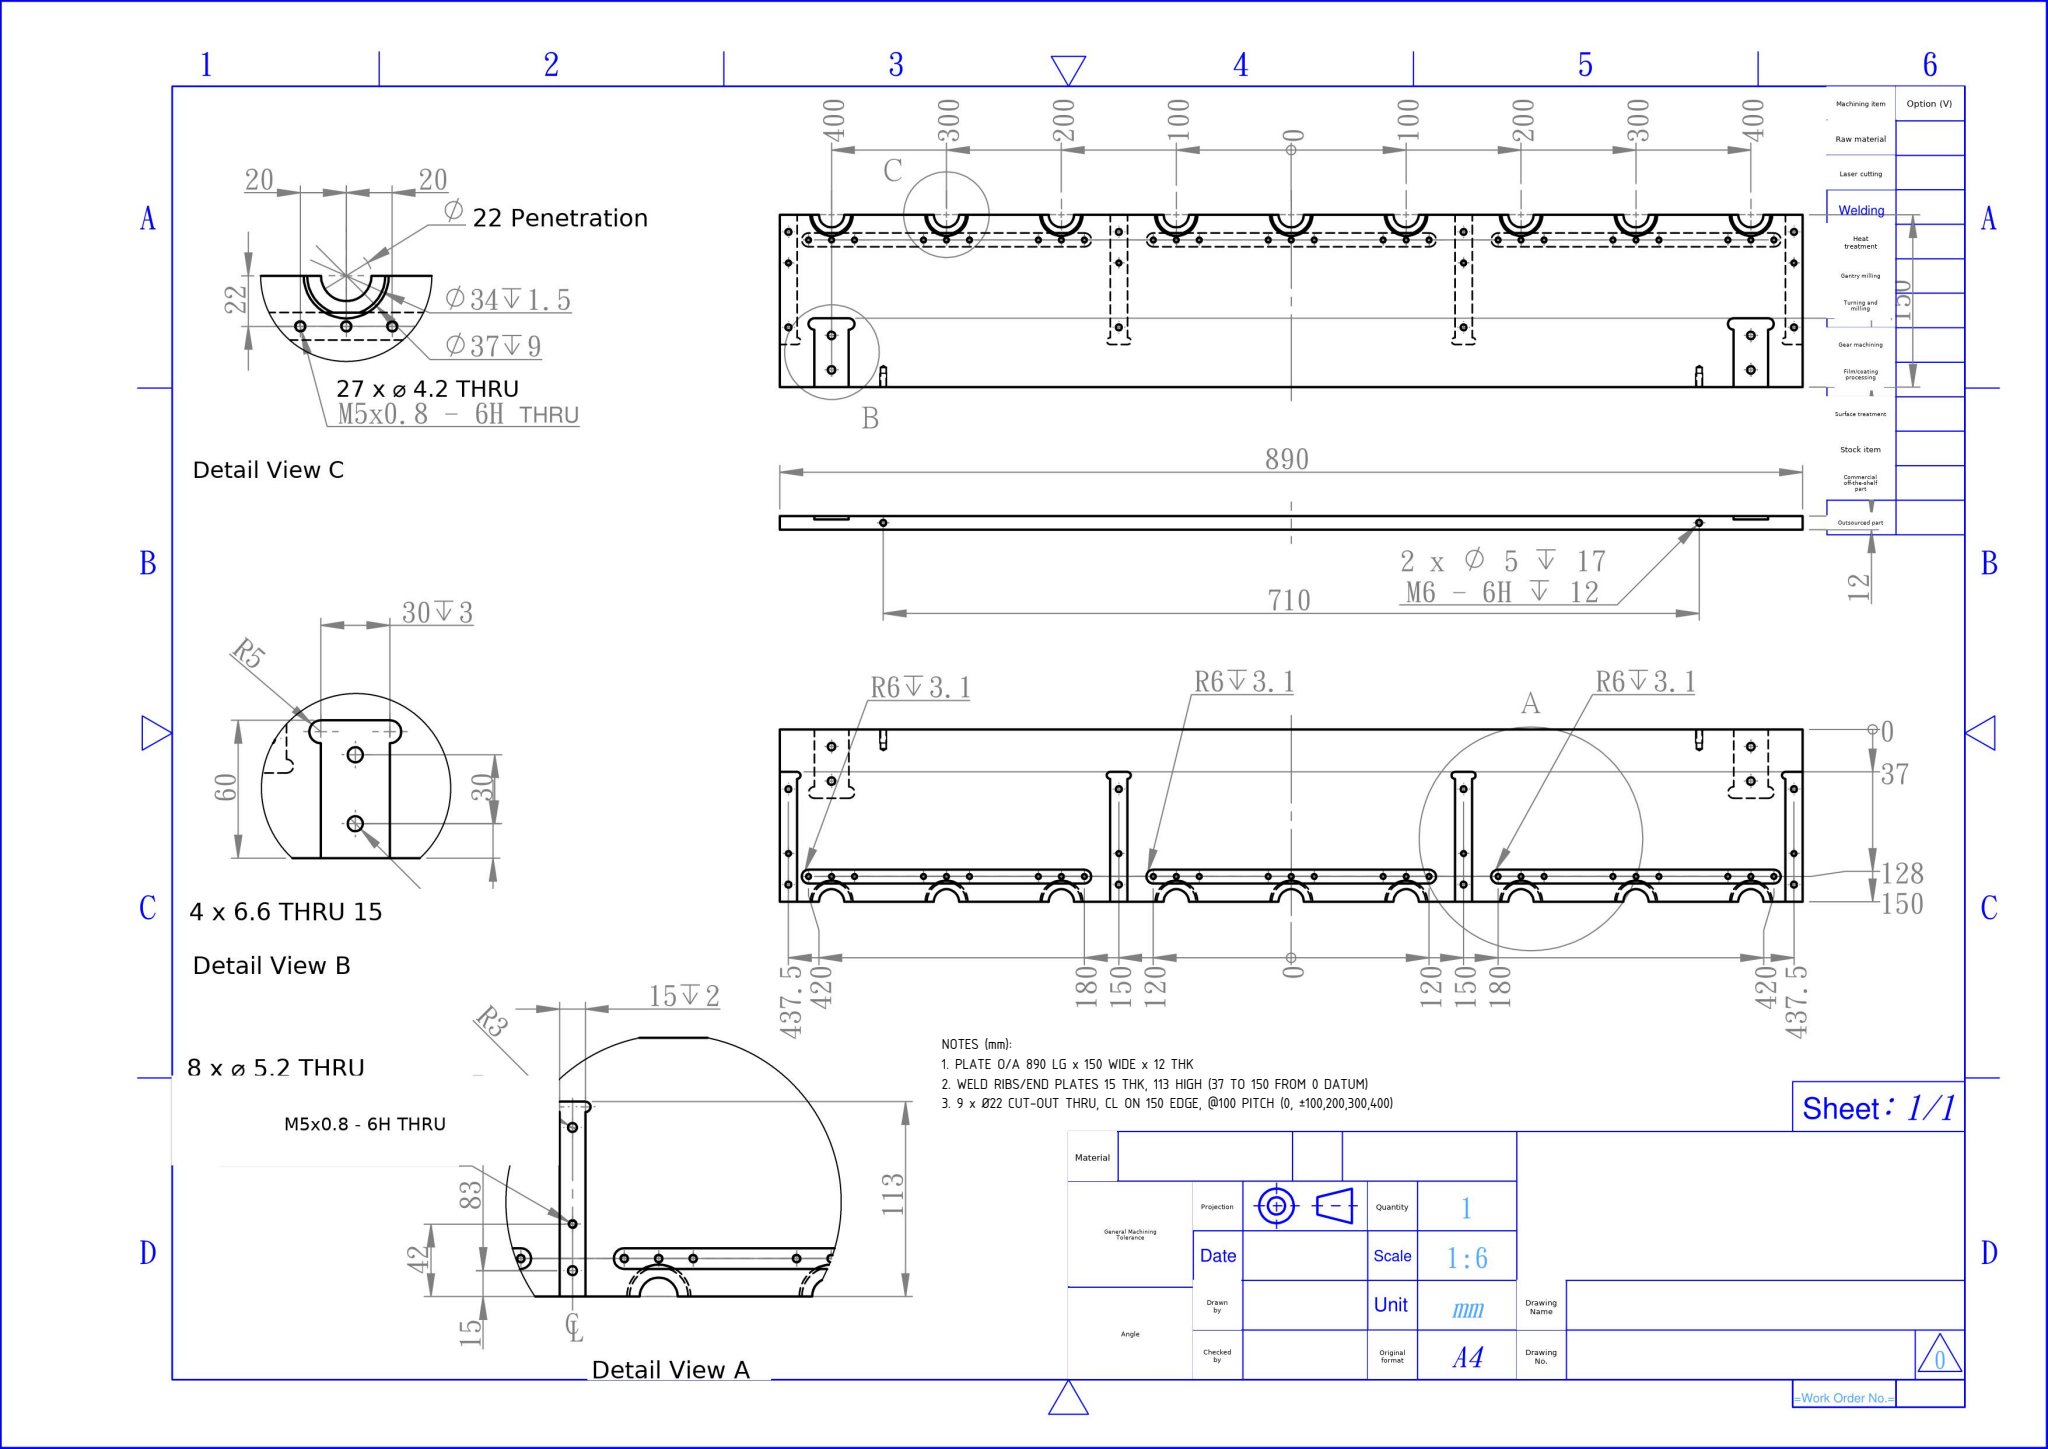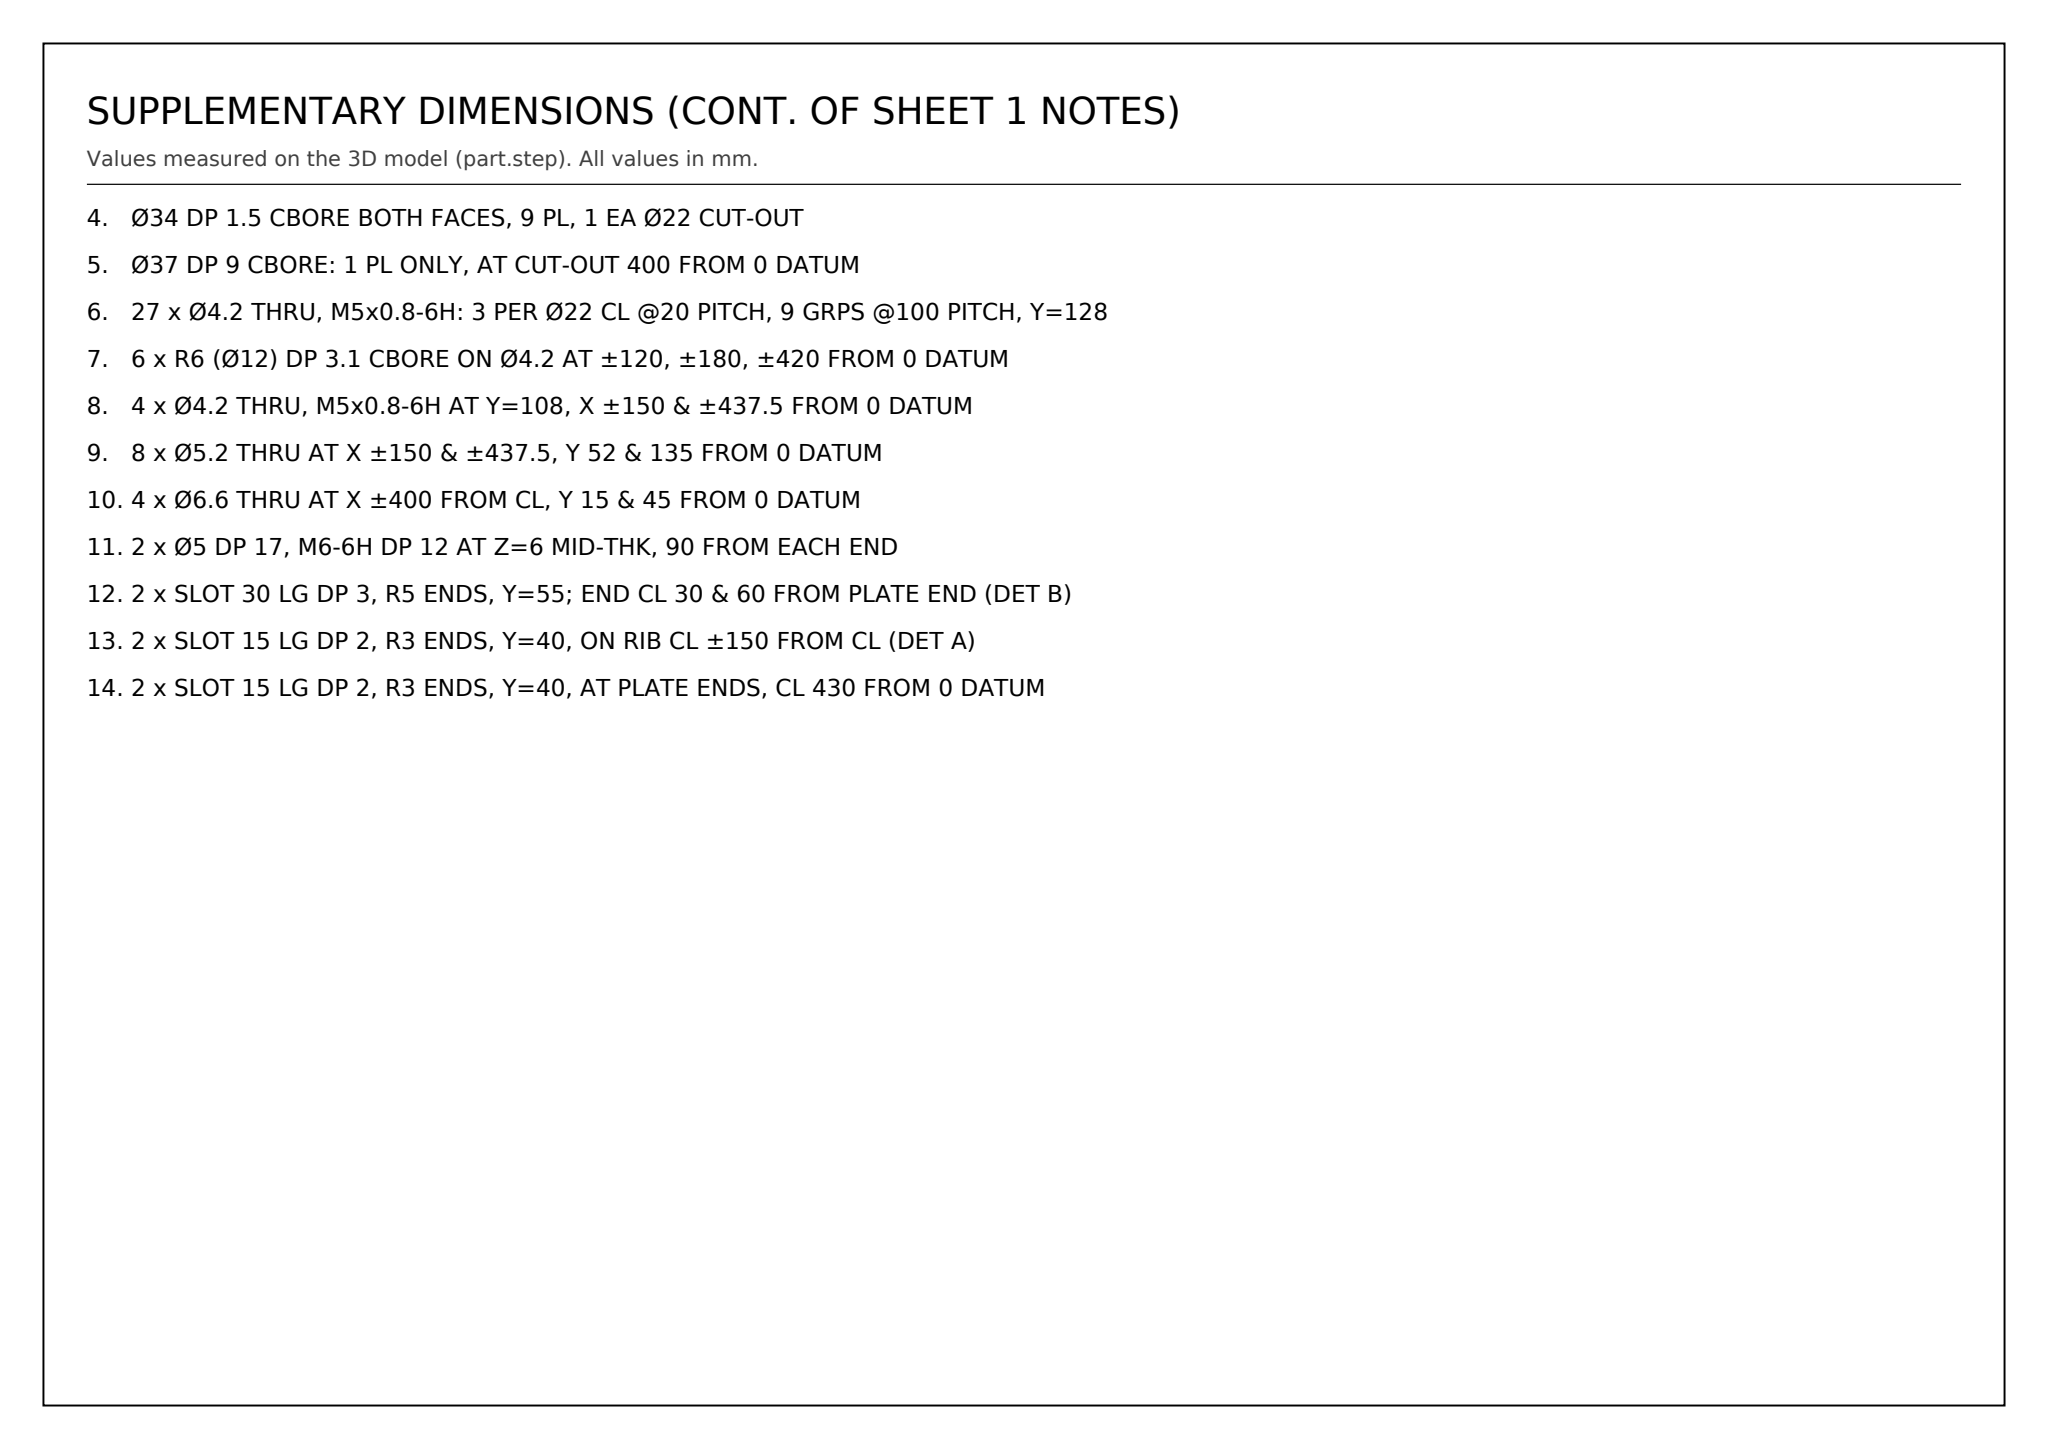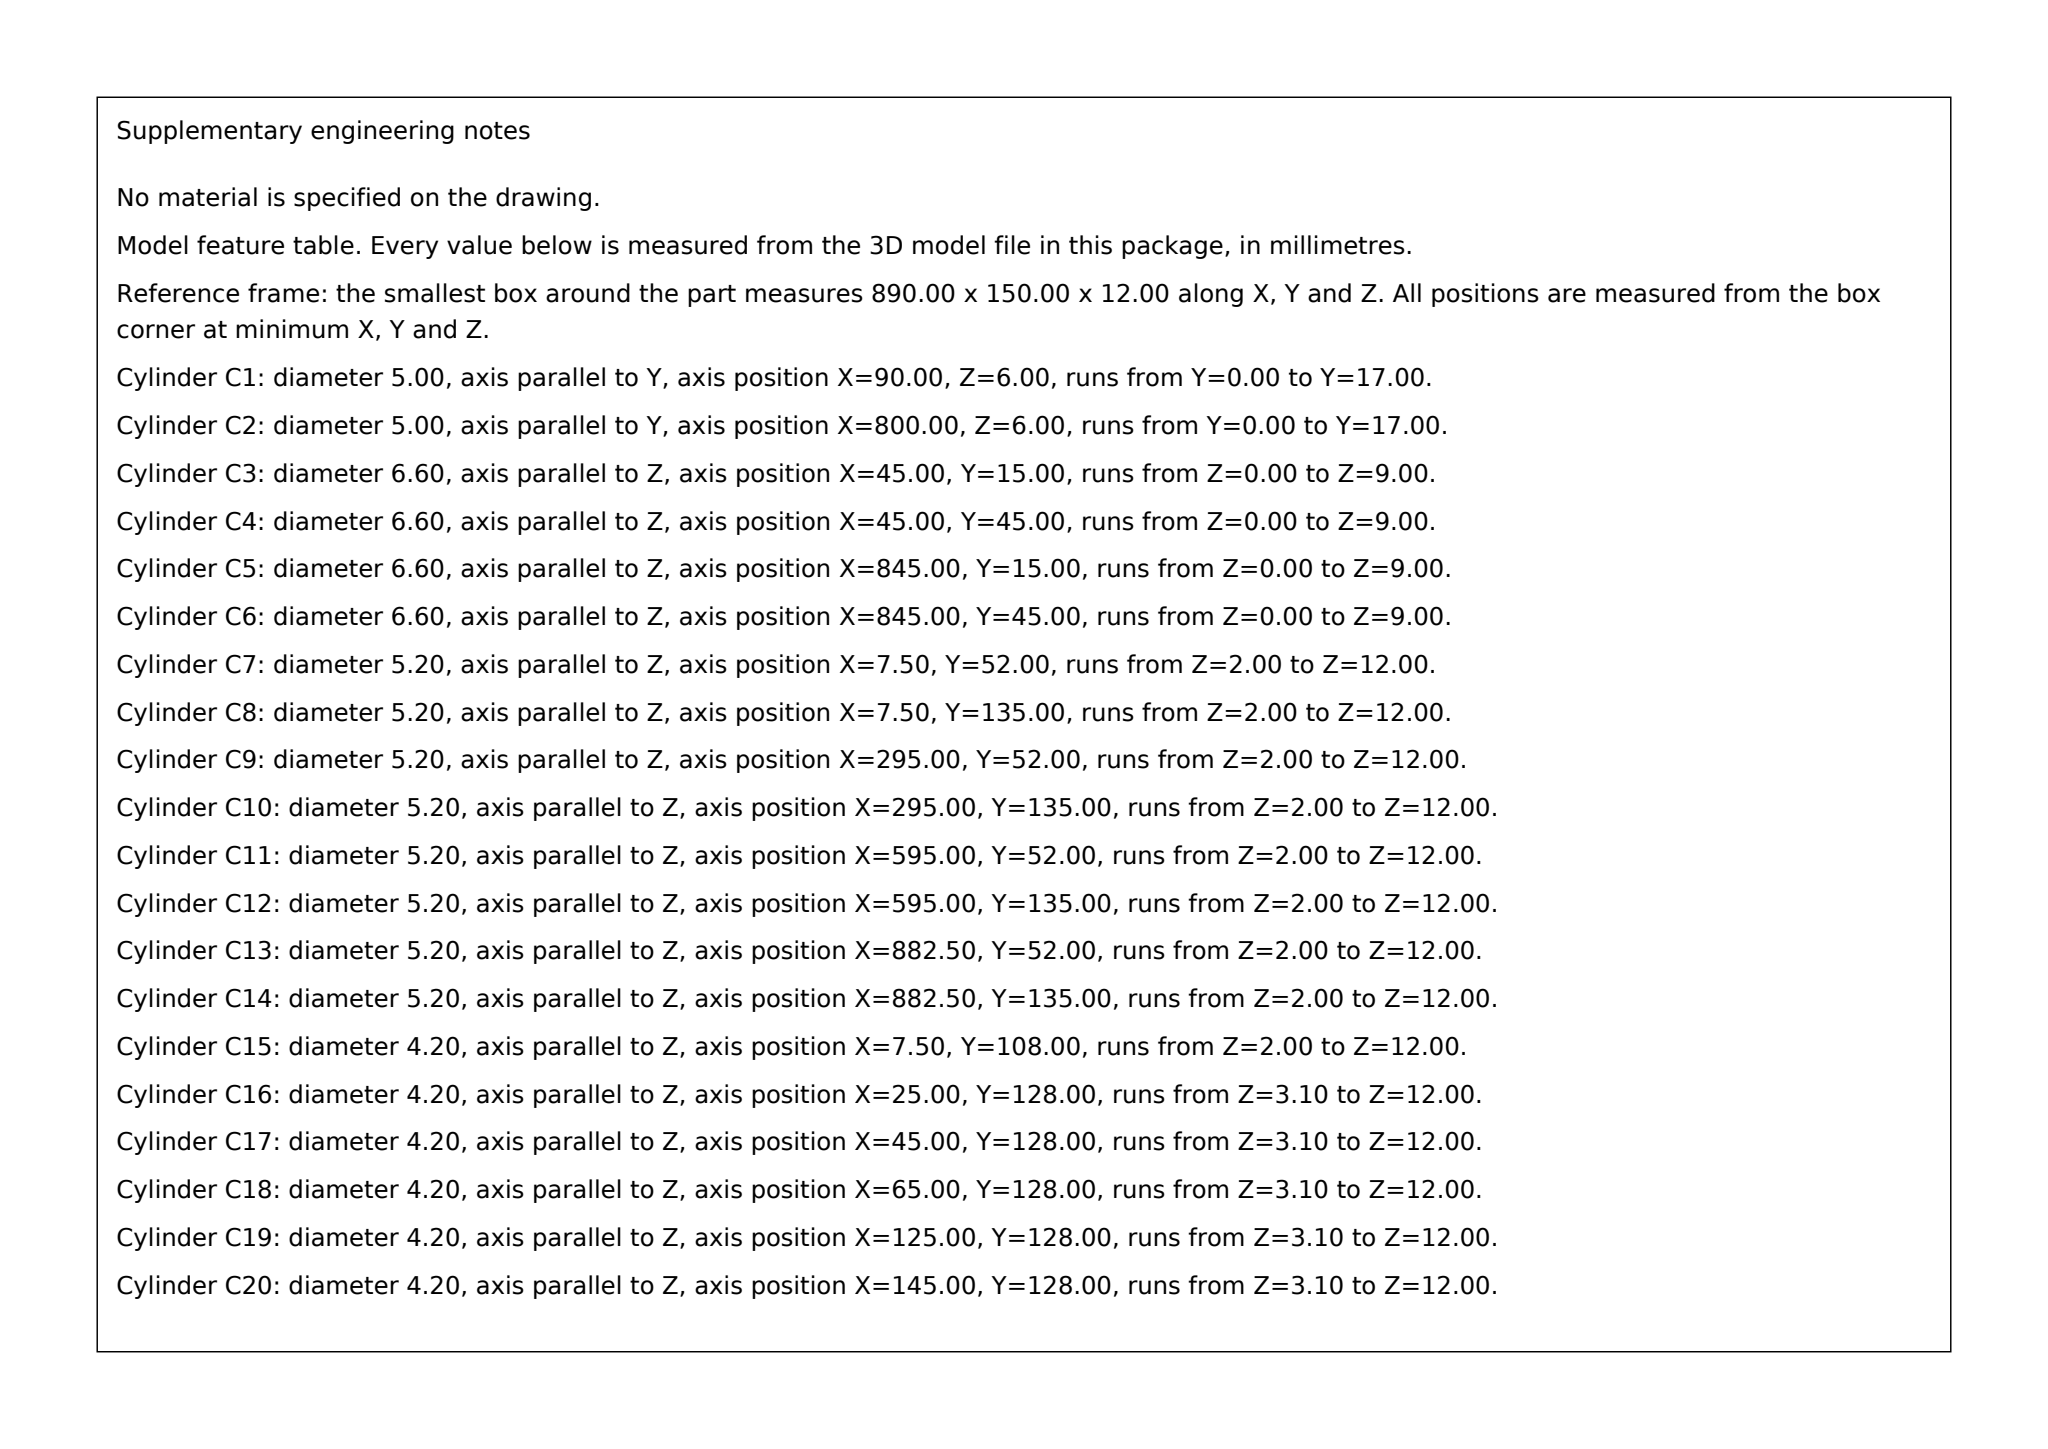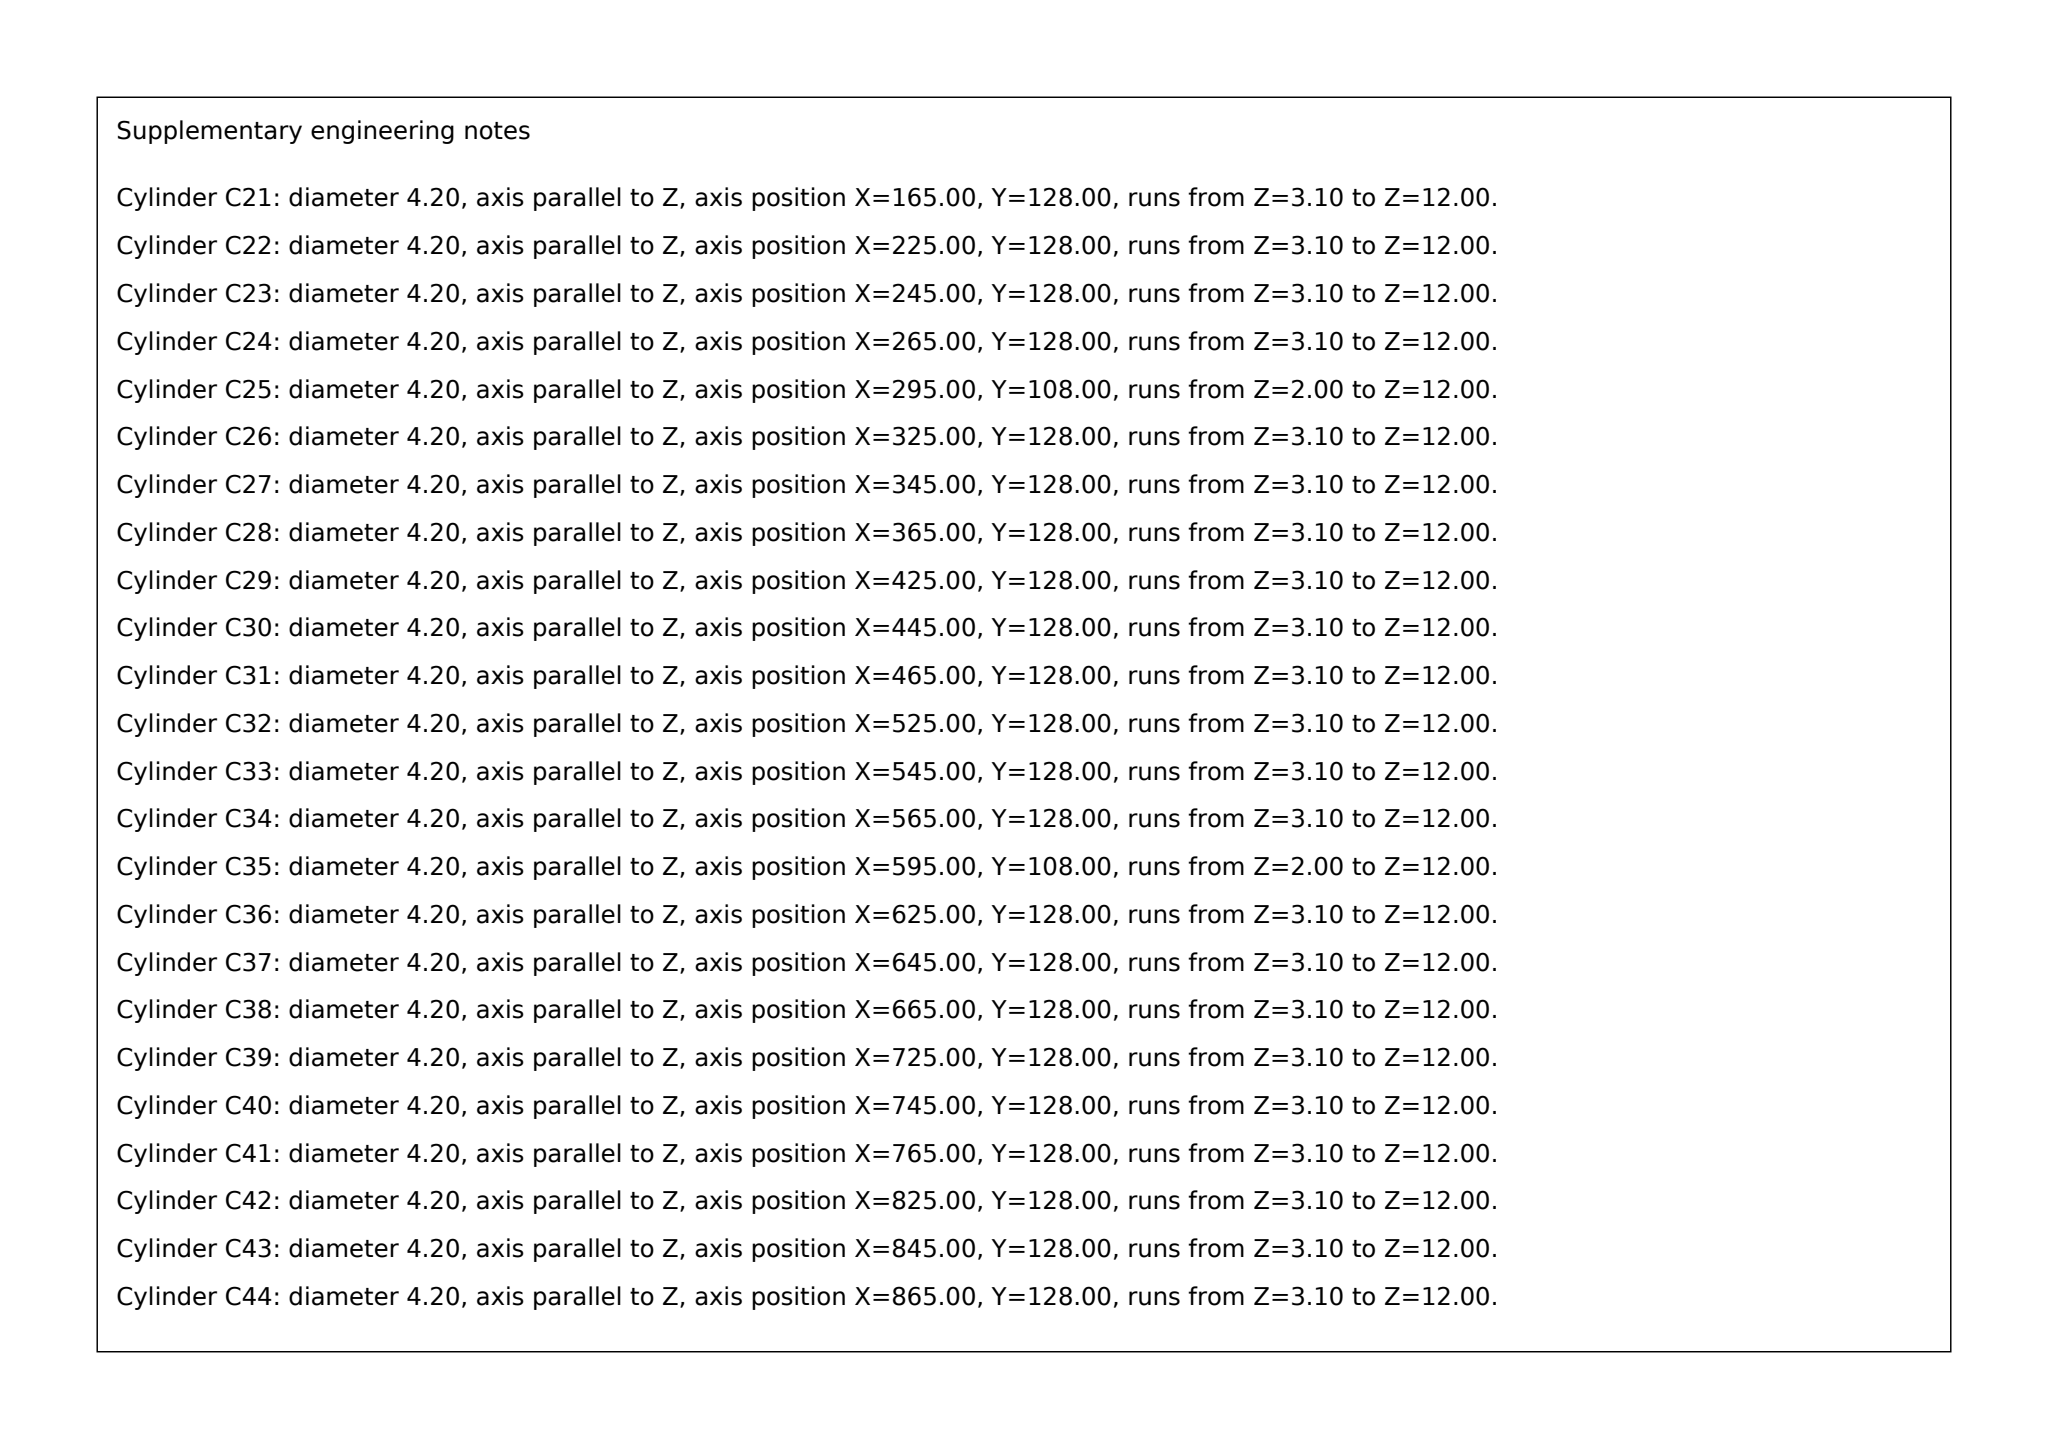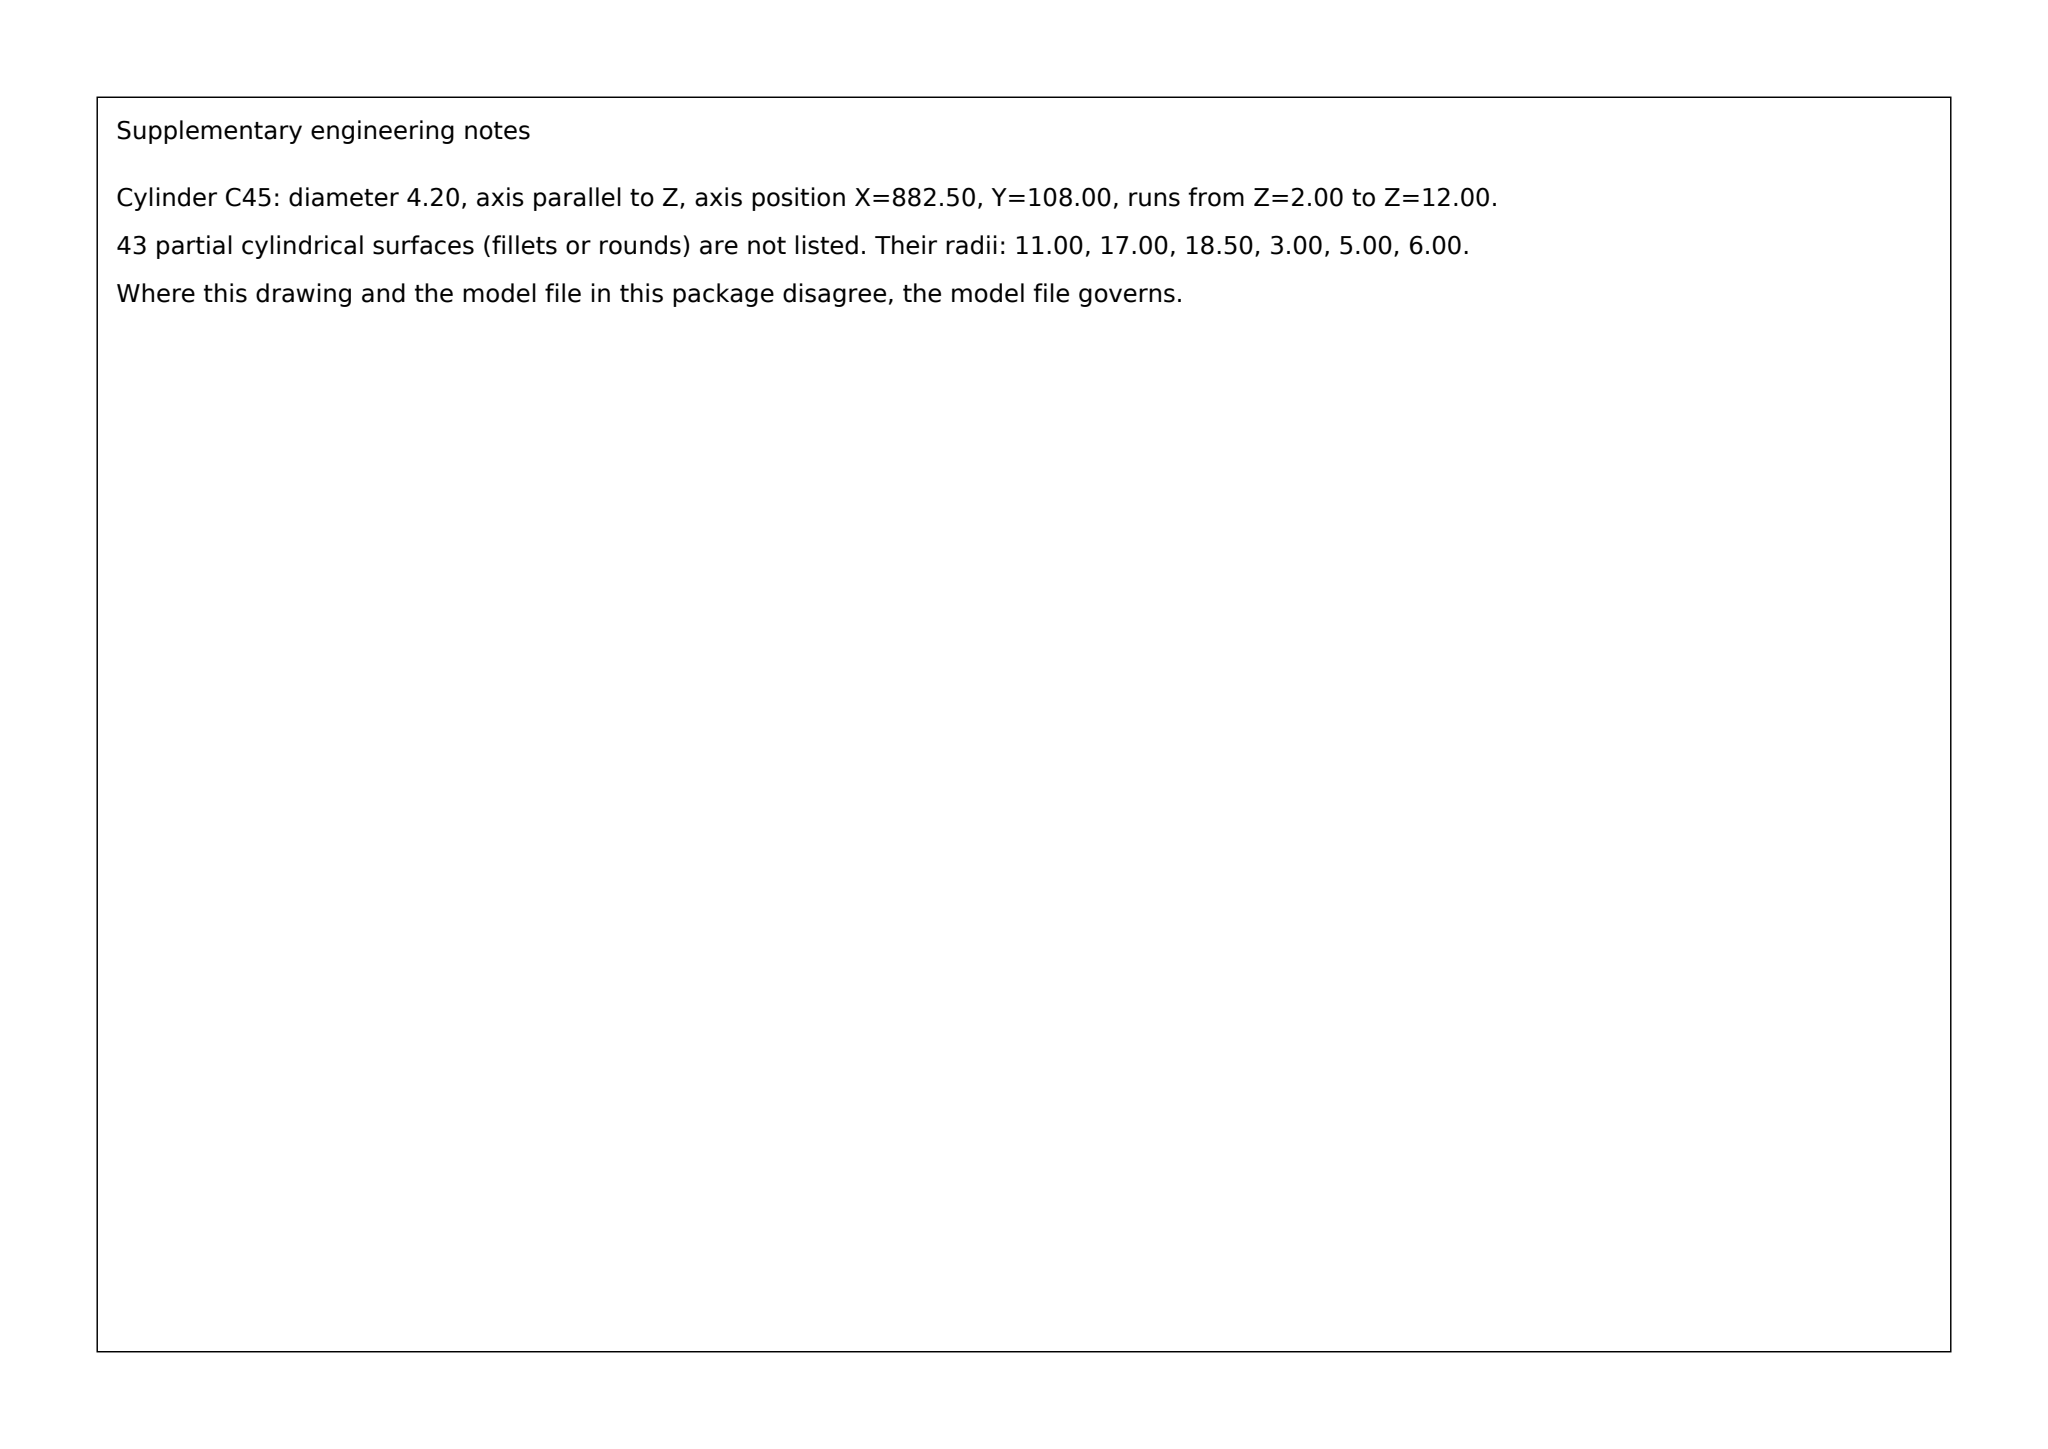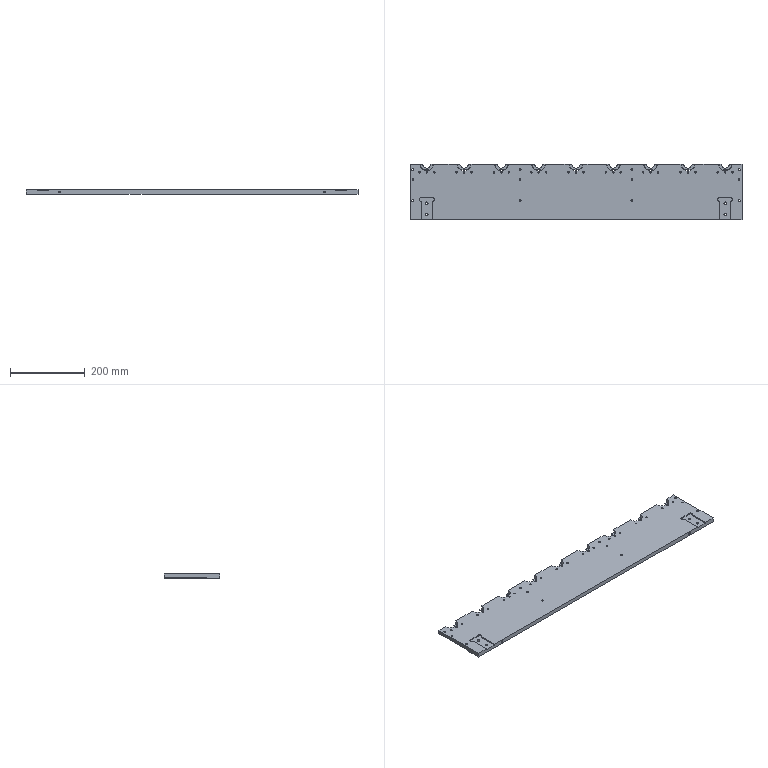Part | SolidWorks | mm | 1 solid | 227 faces | box 890 x 150 x 12 mm | volume 1489554 mm3 | cylinder 150 | plane 73 | cone 4 | commonest cylinder face diameters 4.2 x62 34 x18 5.2 x16 12 x9 6 x9 22 x9 37 x9 6.6 x8
Drawing notes:
PLATE O/A 890 LG x 150 WIDE x 12 THK | from the solid: bbox_xyz = [890.0, 150.0, 12.0]
WELD RIBS/END PLATES 15 THK, 113 HIGH (37 TO 150 FROM 0 DATUM) | from the solid: x-planes 0/15, 287.5/302.5, 587.5/602.5, 875/890 (15 apart); y=37 to y=150 => 113
9 x Ø22 CUT-OUT THRU, CL ON 150 EDGE, @100 PITCH (0, ±100,200,300,400) | from the solid: Ø22/Ø34/Ø37 z-cyls all at y=150.0, x=45..845 @ 100 pitch; CL datum x=445
Ø34 DP 1.5 CBORE BOTH FACES, 9 PL, 1 EA Ø22 CUT-OUT | from the solid: Ø34 dp1.5 count 2 (both faces) at x=45,145,...,845
Ø37 DP 9 CBORE: 1 PL ONLY, AT CUT-OUT 400 FROM 0 DATUM | from the solid: cyl dia 37, axis z, pos [45,150], len 9, count 1; CL x=445 => -400
27 x Ø4.2 THRU, M5x0.8-6H: 3 PER Ø22 CL @20 PITCH, 9 GRPS @100 PITCH, Y=128 | from the solid: Ø4.2 z-holes y=128 at x=25/45/65,125/145/165,...,825/845/865
6 x R6 (Ø12) DP 3.1 CBORE ON Ø4.2 AT ±120, ±180, ±420 FROM 0 DATUM | from the solid: Ø12 dp3.1 cyls at x=25,265,325,565,625,865, y=128; datum x=445
4 x Ø4.2 THRU, M5x0.8-6H AT Y=108, X ±150 & ±437.5 FROM 0 DATUM | from the solid: Ø4.2 len 10 at y=108, x=7.5/295/595/882.5; all other Ø4.2 at y=128
8 x Ø5.2 THRU AT X ±150 & ±437.5, Y 52 & 135 FROM 0 DATUM | from the solid: Ø5.2 z-cyls at x=7.5,295,595,882.5, y=52 & 135
4 x Ø6.6 THRU AT X ±400 FROM CL, Y 15 & 45 FROM 0 DATUM | from the solid: Ø6.6 z-holes at x=45 & 845 (445±400), y=15 & 45, DP 9
2 x Ø5 DP 17, M6-6H DP 12 AT Z=6 MID-THK, 90 FROM EACH END | from the solid: Ø5 y-axis holes at [x=90,z=6] and [x=800,z=6], len 17; 890-800=90
2 x SLOT 30 LG DP 3, R5 ENDS, Y=55; END CL 30 & 60 FROM PLATE END (DET B) | from the solid: Ø10 dp3 ends at x=30/60 and x=830/860, y=55
2 x SLOT 15 LG DP 2, R3 ENDS, Y=40, ON RIB CL ±150 FROM CL (DET A) | from the solid: Ø6 dp2 pairs at x=287.5/302.5 and 587.5/602.5, y=40; rib CLs 295/595
2 x SLOT 15 LG DP 2, R3 ENDS, Y=40, AT PLATE ENDS, CL 430 FROM 0 DATUM | from the solid: Ø6 dp2 at [15,40] and [875,40]; 445-15=430
build123d program:
from build123d import *

# Parameters (mm, degrees)
SKETCH1_W                  = 890
SKETCH1_H                  = 150
BOSS_EXTRUDE1_DEPTH        = 12
CUT_EXTRUDE1_DEPTH         = 3
F_6_6_6_6_DIAMETER_HOLE1_D = 6.6
CUT_EXTRUDE2_REACH         = 453.435
SKETCH5_R                  = 11
SKETCH6_R                  = 17
CUT_EXTRUDE3_DEPTH         = 10.5
SKETCH7_R                  = 18.5
CUT_EXTRUDE5_DEPTH         = 9
M5X0_8_TAPPED_HOLE1_D      = 4.2
LINEAR_PATTERN1_COUNT      = 9
LINEAR_PATTERN1_PITCH      = 100
CUT_EXTRUDE6_DEPTH         = 2
F_5_2_5_2_DIAMETER_HOLE1_D = 5.2
M5X0_8_TAPPED_HOLE2_D      = 4.2
CUT_EXTRUDE7_DEPTH         = 3.1
M6_TAPPED_HOLE1_D          = 5
M6_TAPPED_HOLE1_DEPTH      = 17
M6_TAPPED_HOLE1_TIP        = 1.502


with BuildPart() as part:
    # Sketch1 → Boss-Extrude1 (new body)
    with BuildSketch(Plane.XY):
        Rectangle(SKETCH1_W, SKETCH1_H)
    extrude(amount=BOSS_EXTRUDE1_DEPTH)

    # Sketch2 → Cut-Extrude1 (cut)
    with BuildSketch(Plane.XY.offset(12)):
        with BuildLine():
            Line((-415, -75), (-415, -25))
            ThreePointArc((-415, -25), (-420, -20), (-415, -15))
            Line((-415, -15), (-385, -15))
            ThreePointArc((-385, -15), (-380, -20), (-385, -25))
            Line((-385, -25), (-385, -75))
            Line((-385, -75), (-415, -75))
        make_face()
        with BuildLine():
            Line((385, -25), (385, -75))
            Line((385, -75), (415, -75))
            Line((415, -75), (415, -25))
            ThreePointArc((415, -25), (420, -20), (415, -15))
            Line((415, -15), (385, -15))
            ThreePointArc((385, -15), (380, -20), (385, -25))
        make_face()
    extrude(amount=-CUT_EXTRUDE1_DEPTH, mode=Mode.SUBTRACT)

    # 6.6 _6.6_ Diameter Hole1 (through all)
    with Locations(Plane.XY.offset(9)):
        with Locations((-400, -30), (-400, -60), (400, -60), (400, -30)):
            Hole(F_6_6_6_6_DIAMETER_HOLE1_D / 2)

    # Sketch5 → Cut-Extrude2 (cut, up to next)
    with BuildSketch(Plane.XY.offset(12), mode=Mode.PRIVATE) as cut_extrude2_sk1:
        with Locations((-400, 75)):
            Circle(SKETCH5_R)
    cut_extrude2_tool1 = extrude(cut_extrude2_sk1.sketch, amount=-CUT_EXTRUDE2_REACH, mode=Mode.PRIVATE) & part.part
    cut_extrude2 = cut_extrude2_tool1.solids().sort_by_distance((-400, 75, 12))[0]
    add(cut_extrude2, mode=Mode.SUBTRACT)

    # Sketch6 → Cut-Extrude3 (cut)
    with BuildSketch(Plane.XY.offset(12)):
        with Locations((-400, 75)):
            Circle(SKETCH6_R)
    cut_extrude3 = extrude(amount=-CUT_EXTRUDE3_DEPTH, mode=Mode.SUBTRACT)

    # Sketch7 → Cut-Extrude5 (cut)
    with BuildSketch(Plane.XY.offset(12)):
        with Locations((-400, 75)):
            Circle(SKETCH7_R)
    cut_extrude5 = extrude(amount=-CUT_EXTRUDE5_DEPTH, mode=Mode.SUBTRACT)

    # M5x0.8 Tapped Hole1 (through all)
    with Locations(Plane.XY.offset(12)):
        with Locations((-420, 53), (-400, 53), (-380, 53)):
            m5x0_8_tapped_hole1 = Hole(M5X0_8_TAPPED_HOLE1_D / 2)

    # Linear Pattern1: Cut-Extrude2, Cut-Extrude3, Cut-Extrude5, M5x0.8 Tapped Hole1 ×9
    with Locations(*[(i * LINEAR_PATTERN1_PITCH, 0, 0) for i in range(1, LINEAR_PATTERN1_COUNT)]):
        add(cut_extrude2, mode=Mode.SUBTRACT)
        add(cut_extrude3, mode=Mode.SUBTRACT)
        add(cut_extrude5, mode=Mode.SUBTRACT)
        add(m5x0_8_tapped_hole1, mode=Mode.SUBTRACT)

    # Sketch10 → Cut-Extrude6 (cut)
    with BuildSketch(Plane(origin=(0, 0, 0), x_dir=(-1, 0, 0), z_dir=(0, 0, -1))):
        with BuildLine():
            Line((445, 75), (430, 75))
            Line((430, 75), (430, -32))
            ThreePointArc((430, -32), (427, -35), (430, -38))
            Line((430, -38), (445, -38))
            ThreePointArc((445, -38), (448, -35), (445, -32))
            Line((445, -32), (445, 75))
        make_face()
        with BuildLine():
            Line((-445, 75), (-430, 75))
            Line((-430, 75), (-430, -32))
            ThreePointArc((-430, -32), (-427, -35), (-430, -38))
            Line((-430, -38), (-445, -38))
            ThreePointArc((-445, -38), (-448, -35), (-445, -32))
            Line((-445, -32), (-445, 75))
        make_face()
        with BuildLine():
            Line((-157.5, 75), (-142.5, 75))
            Line((-142.5, 75), (-142.5, -32))
            ThreePointArc((-142.5, -32), (-139.5, -35), (-142.5, -38))
            Line((-142.5, -38), (-157.5, -38))
            ThreePointArc((-157.5, -38), (-160.5, -35), (-157.5, -32))
            Line((-157.5, -32), (-157.5, 75))
        make_face()
        with BuildLine():
            Line((142.5, 75), (157.5, 75))
            Line((157.5, 75), (157.5, -32))
            ThreePointArc((157.5, -32), (160.5, -35), (157.5, -38))
            Line((157.5, -38), (142.5, -38))
            ThreePointArc((142.5, -38), (139.5, -35), (142.5, -32))
            Line((142.5, -32), (142.5, 75))
        make_face()
    extrude(amount=-CUT_EXTRUDE6_DEPTH, mode=Mode.SUBTRACT)

    # 5.2 _5.2_ Diameter Hole1 (through all)
    with Locations(Plane(origin=(0, 0, 2), x_dir=(-1, 0, 0), z_dir=(0, 0, -1))):
        with Locations((437.5, -23), (437.5, 60), (-437.5, 60), (-437.5, -23), (-150, 60), (-150, -23), (150, 60), (150, -23)):
            Hole(F_5_2_5_2_DIAMETER_HOLE1_D / 2)

    # M5x0.8 Tapped Hole2 (through all)
    with Locations(Plane(origin=(0, 0, 2), x_dir=(-1, 0, 0), z_dir=(0, 0, -1))):
        with Locations((437.5, 33), (150, 33), (-150, 33), (-437.5, 33)):
            Hole(M5X0_8_TAPPED_HOLE2_D / 2)

    # Sketch15 → Cut-Extrude7 (cut)
    with BuildSketch(Plane(origin=(0, 0, 0), x_dir=(-1, 0, 0), z_dir=(0, 0, -1))):
        with BuildLine():
            Line((-420, 59), (-180, 59))
            ThreePointArc((-180, 59), (-174, 53), (-180, 47))
            Line((-180, 47), (-420, 47))
            ThreePointArc((-420, 47), (-426, 53), (-420, 59))
        make_face()
        with BuildLine():
            Line((-120, 59), (120, 59))
            ThreePointArc((120, 59), (126, 53), (120, 47))
            Line((120, 47), (-120, 47))
            ThreePointArc((-120, 47), (-126, 53), (-120, 59))
        make_face()
        with BuildLine():
            Line((180, 59), (420, 59))
            ThreePointArc((420, 59), (426, 53), (420, 47))
            Line((420, 47), (180, 47))
            ThreePointArc((180, 47), (174, 53), (180, 59))
        make_face()
    extrude(amount=-CUT_EXTRUDE7_DEPTH, mode=Mode.SUBTRACT)

    # M6 Tapped Hole1
    with Locations(Plane(origin=(0, -75, 0), x_dir=(-1, 0, 0), z_dir=(0, -1, 0))):
        with Locations((355, -6), (-355, -6)):
            Hole(M6_TAPPED_HOLE1_D / 2, depth=M6_TAPPED_HOLE1_DEPTH)
            with Locations((0, 0, -(M6_TAPPED_HOLE1_DEPTH + M6_TAPPED_HOLE1_TIP / 2))):  # 118° drill point
                Cone(0, M6_TAPPED_HOLE1_D / 2, M6_TAPPED_HOLE1_TIP, mode=Mode.SUBTRACT)


solid = part.part